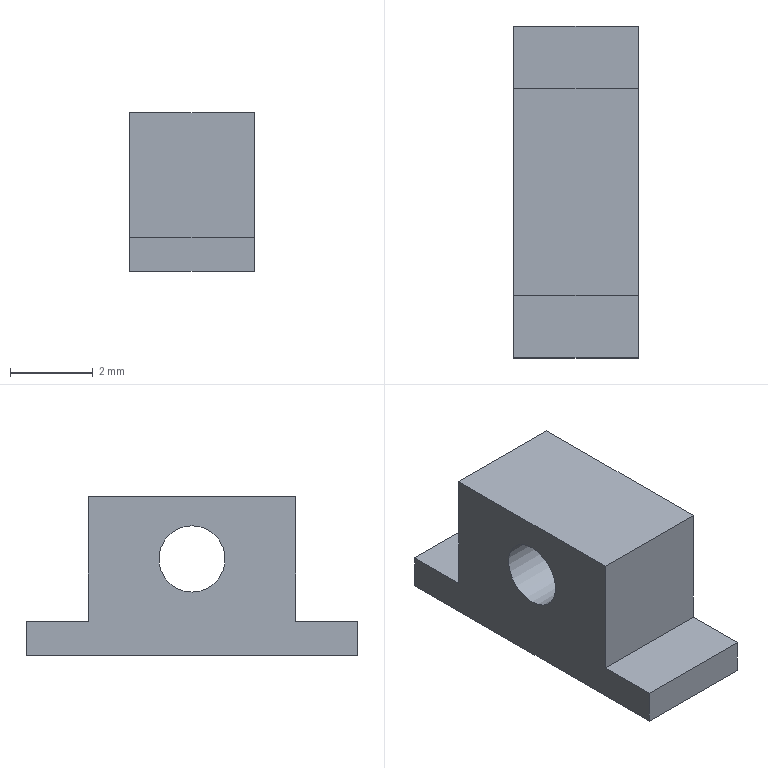Component | NX | LOWER_FIXED_SHAFT | 1 solid | 11 faces | box 3 x 8 x 3.82 mm | volume 59 mm3 | plane 10 | cylinder 1 | commonest cylinder face diameters 1.6 x1
STEP:
#1=CARTESIAN_POINT('',(0.,0.,0.));
#2=DIRECTION('',(0.,0.,1.));
#3=DIRECTION('',(1.,0.,0.));
#4=AXIS2_PLACEMENT_3D('',#1,#2,#3);
#5=CARTESIAN_POINT('',(-42.5,-2.575,4.822));
#6=VERTEX_POINT('',#5);
#7=CARTESIAN_POINT('',(-42.5,-2.575,4.));
#8=VERTEX_POINT('',#7);
#9=CARTESIAN_POINT('',(-42.5,-2.575,4.822));
#10=DIRECTION('',(0.,0.,-1.));
#11=VECTOR('',#10,1.);
#12=LINE('',#9,#11);
#13=CARTESIAN_POINT('',(-34.5,-2.575,4.822));
#14=DIRECTION('',(0.,1.,0.));
#15=DIRECTION('',(0.,0.,1.));
#16=AXIS2_PLACEMENT_3D('',#13,#14,#15);
#17=PLANE('',#16);
#18=CARTESIAN_POINT('',(0.,-8.));
#19=DIRECTION('',(-1.,0.));
#20=VECTOR('',#19,1.);
#21=LINE('',#18,#20);
#22=(GEOMETRIC_REPRESENTATION_CONTEXT(2)PARAMETRIC_REPRESENTATION_CONTEXT()REPRESENTATION_CONTEXT('',''));
#23=DEFINITIONAL_REPRESENTATION('',(#21),#22);
#24=PCURVE('',#17,#23);
#25=CARTESIAN_POINT('',(-42.5,1.425,4.822));
#26=DIRECTION('',(1.,0.,0.));
#27=DIRECTION('',(0.,0.,-1.));
#28=AXIS2_PLACEMENT_3D('',#25,#26,#27);
#29=PLANE('',#28);
#30=CARTESIAN_POINT('',(0.,-4.));
#31=DIRECTION('',(1.,0.));
#32=VECTOR('',#31,1.);
#33=LINE('',#30,#32);
#34=(GEOMETRIC_REPRESENTATION_CONTEXT(2)PARAMETRIC_REPRESENTATION_CONTEXT()REPRESENTATION_CONTEXT('',''));
#35=DEFINITIONAL_REPRESENTATION('',(#33),#34);
#36=PCURVE('',#29,#35);
#37=SURFACE_CURVE('',#12,(#24,#36),.PCURVE_S1.);
#38=EDGE_CURVE('',#6,#8,#37,.T.);
#39=ORIENTED_EDGE('',*,*,#38,.T.);
#40=CARTESIAN_POINT('',(-39.5,-2.575,4.));
#41=VERTEX_POINT('',#40);
#42=CARTESIAN_POINT('',(-34.5,-2.575,4.));
#43=DIRECTION('',(-1.,0.,0.));
#44=VECTOR('',#43,1.);
#45=LINE('',#42,#44);
#46=CARTESIAN_POINT('',(-0.8222,0.));
#47=DIRECTION('',(0.,-1.));
#48=VECTOR('',#47,1.);
#49=LINE('',#46,#48);
#50=(GEOMETRIC_REPRESENTATION_CONTEXT(2)PARAMETRIC_REPRESENTATION_CONTEXT()REPRESENTATION_CONTEXT('',''));
#51=DEFINITIONAL_REPRESENTATION('',(#49),#50);
#52=PCURVE('',#17,#51);
#53=CARTESIAN_POINT('',(-34.5,1.425,4.));
#54=DIRECTION('',(0.,0.,1.));
#55=DIRECTION('',(0.,-1.,0.));
#56=AXIS2_PLACEMENT_3D('',#53,#54,#55);
#57=PLANE('',#56);
#58=CARTESIAN_POINT('',(4.,0.));
#59=DIRECTION('',(0.,-1.));
#60=VECTOR('',#59,1.);
#61=LINE('',#58,#60);
#62=(GEOMETRIC_REPRESENTATION_CONTEXT(2)PARAMETRIC_REPRESENTATION_CONTEXT()REPRESENTATION_CONTEXT('',''));
#63=DEFINITIONAL_REPRESENTATION('',(#61),#62);
#64=PCURVE('',#57,#63);
#65=SURFACE_CURVE('',#45,(#52,#64),.PCURVE_S1.);
#66=EDGE_CURVE('',#41,#8,#65,.T.);
#67=ORIENTED_EDGE('',*,*,#66,.F.);
#68=CARTESIAN_POINT('',(-39.5,-2.575,4.822));
#69=VERTEX_POINT('',#68);
#70=CARTESIAN_POINT('',(-39.5,-2.575,4.822));
#71=DIRECTION('',(0.,0.,-1.));
#72=VECTOR('',#71,1.);
#73=LINE('',#70,#72);
#74=CARTESIAN_POINT('',(0.,-5.));
#75=DIRECTION('',(-1.,0.));
#76=VECTOR('',#75,1.);
#77=LINE('',#74,#76);
#78=(GEOMETRIC_REPRESENTATION_CONTEXT(2)PARAMETRIC_REPRESENTATION_CONTEXT()REPRESENTATION_CONTEXT('',''));
#79=DEFINITIONAL_REPRESENTATION('',(#77),#78);
#80=PCURVE('',#17,#79);
#81=CARTESIAN_POINT('',(-39.5,1.425,4.822));
#82=DIRECTION('',(1.,0.,0.));
#83=DIRECTION('',(0.,0.,-1.));
#84=AXIS2_PLACEMENT_3D('',#81,#82,#83);
#85=PLANE('',#84);
#86=CARTESIAN_POINT('',(0.,-4.));
#87=DIRECTION('',(1.,0.));
#88=VECTOR('',#87,1.);
#89=LINE('',#86,#88);
#90=(GEOMETRIC_REPRESENTATION_CONTEXT(2)PARAMETRIC_REPRESENTATION_CONTEXT()REPRESENTATION_CONTEXT('',''));
#91=DEFINITIONAL_REPRESENTATION('',(#89),#90);
#92=PCURVE('',#85,#91);
#93=SURFACE_CURVE('',#73,(#80,#92),.PCURVE_S1.);
#94=EDGE_CURVE('',#69,#41,#93,.T.);
#95=ORIENTED_EDGE('',*,*,#94,.F.);
#96=CARTESIAN_POINT('',(-34.5,-2.575,4.822));
#97=DIRECTION('',(-1.,0.,0.));
#98=VECTOR('',#97,1.);
#99=LINE('',#96,#98);
#100=CARTESIAN_POINT('',(0.,0.));
#101=DIRECTION('',(0.,-1.));
#102=VECTOR('',#101,1.);
#103=LINE('',#100,#102);
#104=(GEOMETRIC_REPRESENTATION_CONTEXT(2)PARAMETRIC_REPRESENTATION_CONTEXT()REPRESENTATION_CONTEXT('',''));
#105=DEFINITIONAL_REPRESENTATION('',(#103),#104);
#106=PCURVE('',#17,#105);
#107=CARTESIAN_POINT('',(-34.5,-1.075,4.822));
#108=DIRECTION('',(0.,0.,-1.));
#109=DIRECTION('',(0.,1.,0.));
#110=AXIS2_PLACEMENT_3D('',#107,#108,#109);
#111=PLANE('',#110);
#112=CARTESIAN_POINT('',(-1.5,0.));
#113=DIRECTION('',(0.,-1.));
#114=VECTOR('',#113,1.);
#115=LINE('',#112,#114);
#116=(GEOMETRIC_REPRESENTATION_CONTEXT(2)PARAMETRIC_REPRESENTATION_CONTEXT()REPRESENTATION_CONTEXT('',''));
#117=DEFINITIONAL_REPRESENTATION('',(#115),#116);
#118=PCURVE('',#111,#117);
#119=SURFACE_CURVE('',#99,(#106,#118),.PCURVE_S1.);
#120=EDGE_CURVE('',#69,#6,#119,.T.);
#121=ORIENTED_EDGE('',*,*,#120,.T.);
#122=EDGE_LOOP('',(#39,#67,#95,#121));
#123=FACE_BOUND('',#122,.T.);
#124=ADVANCED_FACE('',(#123),#17,.F.);
#125=CARTESIAN_POINT('',(-42.5,5.425,4.));
#126=VERTEX_POINT('',#125);
#127=CARTESIAN_POINT('',(-42.5,1.425,4.));
#128=DIRECTION('',(0.,1.,-0.));
#129=VECTOR('',#128,1.);
#130=LINE('',#127,#129);
#131=CARTESIAN_POINT('',(0.,-8.));
#132=DIRECTION('',(-1.,0.));
#133=VECTOR('',#132,1.);
#134=LINE('',#131,#133);
#135=(GEOMETRIC_REPRESENTATION_CONTEXT(2)PARAMETRIC_REPRESENTATION_CONTEXT()REPRESENTATION_CONTEXT('',''));
#136=DEFINITIONAL_REPRESENTATION('',(#134),#135);
#137=PCURVE('',#57,#136);
#138=CARTESIAN_POINT('',(0.8222,0.));
#139=DIRECTION('',(0.,1.));
#140=VECTOR('',#139,1.);
#141=LINE('',#138,#140);
#142=(GEOMETRIC_REPRESENTATION_CONTEXT(2)PARAMETRIC_REPRESENTATION_CONTEXT()REPRESENTATION_CONTEXT('',''));
#143=DEFINITIONAL_REPRESENTATION('',(#141),#142);
#144=PCURVE('',#29,#143);
#145=SURFACE_CURVE('',#130,(#137,#144),.PCURVE_S1.);
#146=EDGE_CURVE('',#8,#126,#145,.T.);
#147=ORIENTED_EDGE('',*,*,#146,.T.);
#148=CARTESIAN_POINT('',(-39.5,5.425,4.));
#149=VERTEX_POINT('',#148);
#150=CARTESIAN_POINT('',(-34.5,5.425,4.));
#151=DIRECTION('',(-1.,0.,0.));
#152=VECTOR('',#151,1.);
#153=LINE('',#150,#152);
#154=CARTESIAN_POINT('',(-4.,0.));
#155=DIRECTION('',(0.,-1.));
#156=VECTOR('',#155,1.);
#157=LINE('',#154,#156);
#158=(GEOMETRIC_REPRESENTATION_CONTEXT(2)PARAMETRIC_REPRESENTATION_CONTEXT()REPRESENTATION_CONTEXT('',''));
#159=DEFINITIONAL_REPRESENTATION('',(#157),#158);
#160=PCURVE('',#57,#159);
#161=CARTESIAN_POINT('',(-34.5,5.425,3.822));
#162=DIRECTION('',(0.,-1.,0.));
#163=DIRECTION('',(0.,0.,-1.));
#164=AXIS2_PLACEMENT_3D('',#161,#162,#163);
#165=PLANE('',#164);
#166=CARTESIAN_POINT('',(-0.1778,0.));
#167=DIRECTION('',(0.,-1.));
#168=VECTOR('',#167,1.);
#169=LINE('',#166,#168);
#170=(GEOMETRIC_REPRESENTATION_CONTEXT(2)PARAMETRIC_REPRESENTATION_CONTEXT()REPRESENTATION_CONTEXT('',''));
#171=DEFINITIONAL_REPRESENTATION('',(#169),#170);
#172=PCURVE('',#165,#171);
#173=SURFACE_CURVE('',#153,(#160,#172),.PCURVE_S1.);
#174=EDGE_CURVE('',#149,#126,#173,.T.);
#175=ORIENTED_EDGE('',*,*,#174,.F.);
#176=CARTESIAN_POINT('',(-39.5,1.425,4.));
#177=DIRECTION('',(0.,1.,-0.));
#178=VECTOR('',#177,1.);
#179=LINE('',#176,#178);
#180=CARTESIAN_POINT('',(0.,-5.));
#181=DIRECTION('',(-1.,0.));
#182=VECTOR('',#181,1.);
#183=LINE('',#180,#182);
#184=(GEOMETRIC_REPRESENTATION_CONTEXT(2)PARAMETRIC_REPRESENTATION_CONTEXT()REPRESENTATION_CONTEXT('',''));
#185=DEFINITIONAL_REPRESENTATION('',(#183),#184);
#186=PCURVE('',#57,#185);
#187=CARTESIAN_POINT('',(0.8222,0.));
#188=DIRECTION('',(0.,1.));
#189=VECTOR('',#188,1.);
#190=LINE('',#187,#189);
#191=(GEOMETRIC_REPRESENTATION_CONTEXT(2)PARAMETRIC_REPRESENTATION_CONTEXT()REPRESENTATION_CONTEXT('',''));
#192=DEFINITIONAL_REPRESENTATION('',(#190),#191);
#193=PCURVE('',#85,#192);
#194=SURFACE_CURVE('',#179,(#186,#193),.PCURVE_S1.);
#195=EDGE_CURVE('',#41,#149,#194,.T.);
#196=ORIENTED_EDGE('',*,*,#195,.F.);
#197=ORIENTED_EDGE('',*,*,#66,.T.);
#198=EDGE_LOOP('',(#147,#175,#196,#197));
#199=FACE_BOUND('',#198,.T.);
#200=ADVANCED_FACE('',(#199),#57,.F.);
#201=CARTESIAN_POINT('',(-42.5,5.425,4.822));
#202=VERTEX_POINT('',#201);
#203=CARTESIAN_POINT('',(-42.5,5.425,3.822));
#204=DIRECTION('',(0.,0.,1.));
#205=VECTOR('',#204,1.);
#206=LINE('',#203,#205);
#207=CARTESIAN_POINT('',(0.,-8.));
#208=DIRECTION('',(-1.,0.));
#209=VECTOR('',#208,1.);
#210=LINE('',#207,#209);
#211=(GEOMETRIC_REPRESENTATION_CONTEXT(2)PARAMETRIC_REPRESENTATION_CONTEXT()REPRESENTATION_CONTEXT('',''));
#212=DEFINITIONAL_REPRESENTATION('',(#210),#211);
#213=PCURVE('',#165,#212);
#214=CARTESIAN_POINT('',(1.,4.));
#215=DIRECTION('',(-1.,0.));
#216=VECTOR('',#215,1.);
#217=LINE('',#214,#216);
#218=(GEOMETRIC_REPRESENTATION_CONTEXT(2)PARAMETRIC_REPRESENTATION_CONTEXT()REPRESENTATION_CONTEXT('',''));
#219=DEFINITIONAL_REPRESENTATION('',(#217),#218);
#220=PCURVE('',#29,#219);
#221=SURFACE_CURVE('',#206,(#213,#220),.PCURVE_S1.);
#222=EDGE_CURVE('',#126,#202,#221,.T.);
#223=ORIENTED_EDGE('',*,*,#222,.T.);
#224=CARTESIAN_POINT('',(-39.5,5.425,4.822));
#225=VERTEX_POINT('',#224);
#226=CARTESIAN_POINT('',(-34.5,5.425,4.822));
#227=DIRECTION('',(-1.,0.,0.));
#228=VECTOR('',#227,1.);
#229=LINE('',#226,#228);
#230=CARTESIAN_POINT('',(-1.,0.));
#231=DIRECTION('',(0.,-1.));
#232=VECTOR('',#231,1.);
#233=LINE('',#230,#232);
#234=(GEOMETRIC_REPRESENTATION_CONTEXT(2)PARAMETRIC_REPRESENTATION_CONTEXT()REPRESENTATION_CONTEXT('',''));
#235=DEFINITIONAL_REPRESENTATION('',(#233),#234);
#236=PCURVE('',#165,#235);
#237=CARTESIAN_POINT('',(-34.5,5.425,4.822));
#238=DIRECTION('',(0.,-0.,-1.));
#239=DIRECTION('',(0.,1.,-0.));
#240=AXIS2_PLACEMENT_3D('',#237,#238,#239);
#241=PLANE('',#240);
#242=CARTESIAN_POINT('',(0.,0.));
#243=DIRECTION('',(0.,-1.));
#244=VECTOR('',#243,1.);
#245=LINE('',#242,#244);
#246=(GEOMETRIC_REPRESENTATION_CONTEXT(2)PARAMETRIC_REPRESENTATION_CONTEXT()REPRESENTATION_CONTEXT('',''));
#247=DEFINITIONAL_REPRESENTATION('',(#245),#246);
#248=PCURVE('',#241,#247);
#249=SURFACE_CURVE('',#229,(#236,#248),.PCURVE_S1.);
#250=EDGE_CURVE('',#225,#202,#249,.T.);
#251=ORIENTED_EDGE('',*,*,#250,.F.);
#252=CARTESIAN_POINT('',(-39.5,5.425,3.822));
#253=DIRECTION('',(0.,0.,1.));
#254=VECTOR('',#253,1.);
#255=LINE('',#252,#254);
#256=CARTESIAN_POINT('',(0.,-5.));
#257=DIRECTION('',(-1.,0.));
#258=VECTOR('',#257,1.);
#259=LINE('',#256,#258);
#260=(GEOMETRIC_REPRESENTATION_CONTEXT(2)PARAMETRIC_REPRESENTATION_CONTEXT()REPRESENTATION_CONTEXT('',''));
#261=DEFINITIONAL_REPRESENTATION('',(#259),#260);
#262=PCURVE('',#165,#261);
#263=CARTESIAN_POINT('',(1.,4.));
#264=DIRECTION('',(-1.,0.));
#265=VECTOR('',#264,1.);
#266=LINE('',#263,#265);
#267=(GEOMETRIC_REPRESENTATION_CONTEXT(2)PARAMETRIC_REPRESENTATION_CONTEXT()REPRESENTATION_CONTEXT('',''));
#268=DEFINITIONAL_REPRESENTATION('',(#266),#267);
#269=PCURVE('',#85,#268);
#270=SURFACE_CURVE('',#255,(#262,#269),.PCURVE_S1.);
#271=EDGE_CURVE('',#149,#225,#270,.T.);
#272=ORIENTED_EDGE('',*,*,#271,.F.);
#273=ORIENTED_EDGE('',*,*,#174,.T.);
#274=EDGE_LOOP('',(#223,#251,#272,#273));
#275=FACE_BOUND('',#274,.T.);
#276=ADVANCED_FACE('',(#275),#165,.F.);
#277=CARTESIAN_POINT('',(-42.5,3.925,4.822));
#278=VERTEX_POINT('',#277);
#279=CARTESIAN_POINT('',(-42.5,5.425,4.822));
#280=DIRECTION('',(0.,-1.,0.));
#281=VECTOR('',#280,1.);
#282=LINE('',#279,#281);
#283=CARTESIAN_POINT('',(0.,-8.));
#284=DIRECTION('',(-1.,0.));
#285=VECTOR('',#284,1.);
#286=LINE('',#283,#285);
#287=(GEOMETRIC_REPRESENTATION_CONTEXT(2)PARAMETRIC_REPRESENTATION_CONTEXT()REPRESENTATION_CONTEXT('',''));
#288=DEFINITIONAL_REPRESENTATION('',(#286),#287);
#289=PCURVE('',#241,#288);
#290=CARTESIAN_POINT('',(0.,4.));
#291=DIRECTION('',(-0.,-1.));
#292=VECTOR('',#291,1.);
#293=LINE('',#290,#292);
#294=(GEOMETRIC_REPRESENTATION_CONTEXT(2)PARAMETRIC_REPRESENTATION_CONTEXT()REPRESENTATION_CONTEXT('',''));
#295=DEFINITIONAL_REPRESENTATION('',(#293),#294);
#296=PCURVE('',#29,#295);
#297=SURFACE_CURVE('',#282,(#289,#296),.PCURVE_S1.);
#298=EDGE_CURVE('',#202,#278,#297,.T.);
#299=ORIENTED_EDGE('',*,*,#298,.T.);
#300=CARTESIAN_POINT('',(-39.5,3.925,4.822));
#301=VERTEX_POINT('',#300);
#302=CARTESIAN_POINT('',(-34.5,3.925,4.822));
#303=DIRECTION('',(-1.,0.,0.));
#304=VECTOR('',#303,1.);
#305=LINE('',#302,#304);
#306=CARTESIAN_POINT('',(-1.5,0.));
#307=DIRECTION('',(0.,-1.));
#308=VECTOR('',#307,1.);
#309=LINE('',#306,#308);
#310=(GEOMETRIC_REPRESENTATION_CONTEXT(2)PARAMETRIC_REPRESENTATION_CONTEXT()REPRESENTATION_CONTEXT('',''));
#311=DEFINITIONAL_REPRESENTATION('',(#309),#310);
#312=PCURVE('',#241,#311);
#313=CARTESIAN_POINT('',(-34.5,3.925,4.822));
#314=DIRECTION('',(0.,-1.,0.));
#315=DIRECTION('',(0.,0.,-1.));
#316=AXIS2_PLACEMENT_3D('',#313,#314,#315);
#317=PLANE('',#316);
#318=CARTESIAN_POINT('',(0.,0.));
#319=DIRECTION('',(0.,-1.));
#320=VECTOR('',#319,1.);
#321=LINE('',#318,#320);
#322=(GEOMETRIC_REPRESENTATION_CONTEXT(2)PARAMETRIC_REPRESENTATION_CONTEXT()REPRESENTATION_CONTEXT('',''));
#323=DEFINITIONAL_REPRESENTATION('',(#321),#322);
#324=PCURVE('',#317,#323);
#325=SURFACE_CURVE('',#305,(#312,#324),.PCURVE_S1.);
#326=EDGE_CURVE('',#301,#278,#325,.T.);
#327=ORIENTED_EDGE('',*,*,#326,.F.);
#328=CARTESIAN_POINT('',(-39.5,5.425,4.822));
#329=DIRECTION('',(0.,-1.,0.));
#330=VECTOR('',#329,1.);
#331=LINE('',#328,#330);
#332=CARTESIAN_POINT('',(0.,-5.));
#333=DIRECTION('',(-1.,0.));
#334=VECTOR('',#333,1.);
#335=LINE('',#332,#334);
#336=(GEOMETRIC_REPRESENTATION_CONTEXT(2)PARAMETRIC_REPRESENTATION_CONTEXT()REPRESENTATION_CONTEXT('',''));
#337=DEFINITIONAL_REPRESENTATION('',(#335),#336);
#338=PCURVE('',#241,#337);
#339=CARTESIAN_POINT('',(0.,4.));
#340=DIRECTION('',(-0.,-1.));
#341=VECTOR('',#340,1.);
#342=LINE('',#339,#341);
#343=(GEOMETRIC_REPRESENTATION_CONTEXT(2)PARAMETRIC_REPRESENTATION_CONTEXT()REPRESENTATION_CONTEXT('',''));
#344=DEFINITIONAL_REPRESENTATION('',(#342),#343);
#345=PCURVE('',#85,#344);
#346=SURFACE_CURVE('',#331,(#338,#345),.PCURVE_S1.);
#347=EDGE_CURVE('',#225,#301,#346,.T.);
#348=ORIENTED_EDGE('',*,*,#347,.F.);
#349=ORIENTED_EDGE('',*,*,#250,.T.);
#350=EDGE_LOOP('',(#299,#327,#348,#349));
#351=FACE_BOUND('',#350,.T.);
#352=ADVANCED_FACE('',(#351),#241,.F.);
#353=CARTESIAN_POINT('',(-42.5,3.925,7.822));
#354=VERTEX_POINT('',#353);
#355=CARTESIAN_POINT('',(-42.5,3.925,4.822));
#356=DIRECTION('',(0.,0.,1.));
#357=VECTOR('',#356,1.);
#358=LINE('',#355,#357);
#359=CARTESIAN_POINT('',(0.,-8.));
#360=DIRECTION('',(-1.,0.));
#361=VECTOR('',#360,1.);
#362=LINE('',#359,#361);
#363=(GEOMETRIC_REPRESENTATION_CONTEXT(2)PARAMETRIC_REPRESENTATION_CONTEXT()REPRESENTATION_CONTEXT('',''));
#364=DEFINITIONAL_REPRESENTATION('',(#362),#363);
#365=PCURVE('',#317,#364);
#366=CARTESIAN_POINT('',(0.,2.5));
#367=DIRECTION('',(-1.,0.));
#368=VECTOR('',#367,1.);
#369=LINE('',#366,#368);
#370=(GEOMETRIC_REPRESENTATION_CONTEXT(2)PARAMETRIC_REPRESENTATION_CONTEXT()REPRESENTATION_CONTEXT('',''));
#371=DEFINITIONAL_REPRESENTATION('',(#369),#370);
#372=PCURVE('',#29,#371);
#373=SURFACE_CURVE('',#358,(#365,#372),.PCURVE_S1.);
#374=EDGE_CURVE('',#278,#354,#373,.T.);
#375=ORIENTED_EDGE('',*,*,#374,.T.);
#376=CARTESIAN_POINT('',(-39.5,3.925,7.822));
#377=VERTEX_POINT('',#376);
#378=CARTESIAN_POINT('',(-34.5,3.925,7.822));
#379=DIRECTION('',(-1.,0.,0.));
#380=VECTOR('',#379,1.);
#381=LINE('',#378,#380);
#382=CARTESIAN_POINT('',(-3.,0.));
#383=DIRECTION('',(0.,-1.));
#384=VECTOR('',#383,1.);
#385=LINE('',#382,#384);
#386=(GEOMETRIC_REPRESENTATION_CONTEXT(2)PARAMETRIC_REPRESENTATION_CONTEXT()REPRESENTATION_CONTEXT('',''));
#387=DEFINITIONAL_REPRESENTATION('',(#385),#386);
#388=PCURVE('',#317,#387);
#389=CARTESIAN_POINT('',(-34.5,1.425,7.822));
#390=DIRECTION('',(0.,0.,-1.));
#391=DIRECTION('',(0.,1.,0.));
#392=AXIS2_PLACEMENT_3D('',#389,#390,#391);
#393=PLANE('',#392);
#394=CARTESIAN_POINT('',(2.5,0.));
#395=DIRECTION('',(0.,-1.));
#396=VECTOR('',#395,1.);
#397=LINE('',#394,#396);
#398=(GEOMETRIC_REPRESENTATION_CONTEXT(2)PARAMETRIC_REPRESENTATION_CONTEXT()REPRESENTATION_CONTEXT('',''));
#399=DEFINITIONAL_REPRESENTATION('',(#397),#398);
#400=PCURVE('',#393,#399);
#401=SURFACE_CURVE('',#381,(#388,#400),.PCURVE_S1.);
#402=EDGE_CURVE('',#377,#354,#401,.T.);
#403=ORIENTED_EDGE('',*,*,#402,.F.);
#404=CARTESIAN_POINT('',(-39.5,3.925,4.822));
#405=DIRECTION('',(0.,0.,1.));
#406=VECTOR('',#405,1.);
#407=LINE('',#404,#406);
#408=CARTESIAN_POINT('',(0.,-5.));
#409=DIRECTION('',(-1.,0.));
#410=VECTOR('',#409,1.);
#411=LINE('',#408,#410);
#412=(GEOMETRIC_REPRESENTATION_CONTEXT(2)PARAMETRIC_REPRESENTATION_CONTEXT()REPRESENTATION_CONTEXT('',''));
#413=DEFINITIONAL_REPRESENTATION('',(#411),#412);
#414=PCURVE('',#317,#413);
#415=CARTESIAN_POINT('',(0.,2.5));
#416=DIRECTION('',(-1.,0.));
#417=VECTOR('',#416,1.);
#418=LINE('',#415,#417);
#419=(GEOMETRIC_REPRESENTATION_CONTEXT(2)PARAMETRIC_REPRESENTATION_CONTEXT()REPRESENTATION_CONTEXT('',''));
#420=DEFINITIONAL_REPRESENTATION('',(#418),#419);
#421=PCURVE('',#85,#420);
#422=SURFACE_CURVE('',#407,(#414,#421),.PCURVE_S1.);
#423=EDGE_CURVE('',#301,#377,#422,.T.);
#424=ORIENTED_EDGE('',*,*,#423,.F.);
#425=ORIENTED_EDGE('',*,*,#326,.T.);
#426=EDGE_LOOP('',(#375,#403,#424,#425));
#427=FACE_BOUND('',#426,.T.);
#428=ADVANCED_FACE('',(#427),#317,.F.);
#429=CARTESIAN_POINT('',(-42.5,-1.075,7.822));
#430=VERTEX_POINT('',#429);
#431=CARTESIAN_POINT('',(-42.5,1.425,7.822));
#432=DIRECTION('',(0.,-1.,-0.));
#433=VECTOR('',#432,1.);
#434=LINE('',#431,#433);
#435=CARTESIAN_POINT('',(0.,-8.));
#436=DIRECTION('',(-1.,0.));
#437=VECTOR('',#436,1.);
#438=LINE('',#435,#437);
#439=(GEOMETRIC_REPRESENTATION_CONTEXT(2)PARAMETRIC_REPRESENTATION_CONTEXT()REPRESENTATION_CONTEXT('',''));
#440=DEFINITIONAL_REPRESENTATION('',(#438),#439);
#441=PCURVE('',#393,#440);
#442=CARTESIAN_POINT('',(-3.,0.));
#443=DIRECTION('',(0.,-1.));
#444=VECTOR('',#443,1.);
#445=LINE('',#442,#444);
#446=(GEOMETRIC_REPRESENTATION_CONTEXT(2)PARAMETRIC_REPRESENTATION_CONTEXT()REPRESENTATION_CONTEXT('',''));
#447=DEFINITIONAL_REPRESENTATION('',(#445),#446);
#448=PCURVE('',#29,#447);
#449=SURFACE_CURVE('',#434,(#441,#448),.PCURVE_S1.);
#450=EDGE_CURVE('',#354,#430,#449,.T.);
#451=ORIENTED_EDGE('',*,*,#450,.T.);
#452=CARTESIAN_POINT('',(-39.5,-1.075,7.822));
#453=VERTEX_POINT('',#452);
#454=CARTESIAN_POINT('',(-34.5,-1.075,7.822));
#455=DIRECTION('',(-1.,0.,0.));
#456=VECTOR('',#455,1.);
#457=LINE('',#454,#456);
#458=CARTESIAN_POINT('',(-2.5,0.));
#459=DIRECTION('',(0.,-1.));
#460=VECTOR('',#459,1.);
#461=LINE('',#458,#460);
#462=(GEOMETRIC_REPRESENTATION_CONTEXT(2)PARAMETRIC_REPRESENTATION_CONTEXT()REPRESENTATION_CONTEXT('',''));
#463=DEFINITIONAL_REPRESENTATION('',(#461),#462);
#464=PCURVE('',#393,#463);
#465=CARTESIAN_POINT('',(-34.5,-1.075,7.822));
#466=DIRECTION('',(0.,1.,0.));
#467=DIRECTION('',(0.,0.,1.));
#468=AXIS2_PLACEMENT_3D('',#465,#466,#467);
#469=PLANE('',#468);
#470=CARTESIAN_POINT('',(0.,0.));
#471=DIRECTION('',(0.,-1.));
#472=VECTOR('',#471,1.);
#473=LINE('',#470,#472);
#474=(GEOMETRIC_REPRESENTATION_CONTEXT(2)PARAMETRIC_REPRESENTATION_CONTEXT()REPRESENTATION_CONTEXT('',''));
#475=DEFINITIONAL_REPRESENTATION('',(#473),#474);
#476=PCURVE('',#469,#475);
#477=SURFACE_CURVE('',#457,(#464,#476),.PCURVE_S1.);
#478=EDGE_CURVE('',#453,#430,#477,.T.);
#479=ORIENTED_EDGE('',*,*,#478,.F.);
#480=CARTESIAN_POINT('',(-39.5,3.925,7.822));
#481=DIRECTION('',(0.,-1.,0.));
#482=VECTOR('',#481,1.);
#483=LINE('',#480,#482);
#484=CARTESIAN_POINT('',(2.5,-5.));
#485=DIRECTION('',(-1.,0.));
#486=VECTOR('',#485,1.);
#487=LINE('',#484,#486);
#488=(GEOMETRIC_REPRESENTATION_CONTEXT(2)PARAMETRIC_REPRESENTATION_CONTEXT()REPRESENTATION_CONTEXT('',''));
#489=DEFINITIONAL_REPRESENTATION('',(#487),#488);
#490=PCURVE('',#393,#489);
#491=CARTESIAN_POINT('',(-3.,2.5));
#492=DIRECTION('',(-0.,-1.));
#493=VECTOR('',#492,1.);
#494=LINE('',#491,#493);
#495=(GEOMETRIC_REPRESENTATION_CONTEXT(2)PARAMETRIC_REPRESENTATION_CONTEXT()REPRESENTATION_CONTEXT('',''));
#496=DEFINITIONAL_REPRESENTATION('',(#494),#495);
#497=PCURVE('',#85,#496);
#498=SURFACE_CURVE('',#483,(#490,#497),.PCURVE_S1.);
#499=EDGE_CURVE('',#377,#453,#498,.T.);
#500=ORIENTED_EDGE('',*,*,#499,.F.);
#501=ORIENTED_EDGE('',*,*,#402,.T.);
#502=EDGE_LOOP('',(#451,#479,#500,#501));
#503=FACE_BOUND('',#502,.T.);
#504=ADVANCED_FACE('',(#503),#393,.F.);
#505=CARTESIAN_POINT('',(-42.5,-1.075,4.822));
#506=VERTEX_POINT('',#505);
#507=CARTESIAN_POINT('',(-42.5,-1.075,7.822));
#508=DIRECTION('',(0.,0.,-1.));
#509=VECTOR('',#508,1.);
#510=LINE('',#507,#509);
#511=CARTESIAN_POINT('',(0.,-8.));
#512=DIRECTION('',(-1.,0.));
#513=VECTOR('',#512,1.);
#514=LINE('',#511,#513);
#515=(GEOMETRIC_REPRESENTATION_CONTEXT(2)PARAMETRIC_REPRESENTATION_CONTEXT()REPRESENTATION_CONTEXT('',''));
#516=DEFINITIONAL_REPRESENTATION('',(#514),#515);
#517=PCURVE('',#469,#516);
#518=CARTESIAN_POINT('',(-3.,-2.5));
#519=DIRECTION('',(1.,0.));
#520=VECTOR('',#519,1.);
#521=LINE('',#518,#520);
#522=(GEOMETRIC_REPRESENTATION_CONTEXT(2)PARAMETRIC_REPRESENTATION_CONTEXT()REPRESENTATION_CONTEXT('',''));
#523=DEFINITIONAL_REPRESENTATION('',(#521),#522);
#524=PCURVE('',#29,#523);
#525=SURFACE_CURVE('',#510,(#517,#524),.PCURVE_S1.);
#526=EDGE_CURVE('',#430,#506,#525,.T.);
#527=ORIENTED_EDGE('',*,*,#526,.T.);
#528=CARTESIAN_POINT('',(-39.5,-1.075,4.822));
#529=VERTEX_POINT('',#528);
#530=CARTESIAN_POINT('',(-34.5,-1.075,4.822));
#531=DIRECTION('',(-1.,0.,0.));
#532=VECTOR('',#531,1.);
#533=LINE('',#530,#532);
#534=CARTESIAN_POINT('',(-3.,0.));
#535=DIRECTION('',(0.,-1.));
#536=VECTOR('',#535,1.);
#537=LINE('',#534,#536);
#538=(GEOMETRIC_REPRESENTATION_CONTEXT(2)PARAMETRIC_REPRESENTATION_CONTEXT()REPRESENTATION_CONTEXT('',''));
#539=DEFINITIONAL_REPRESENTATION('',(#537),#538);
#540=PCURVE('',#469,#539);
#541=CARTESIAN_POINT('',(0.,0.));
#542=DIRECTION('',(0.,-1.));
#543=VECTOR('',#542,1.);
#544=LINE('',#541,#543);
#545=(GEOMETRIC_REPRESENTATION_CONTEXT(2)PARAMETRIC_REPRESENTATION_CONTEXT()REPRESENTATION_CONTEXT('',''));
#546=DEFINITIONAL_REPRESENTATION('',(#544),#545);
#547=PCURVE('',#111,#546);
#548=SURFACE_CURVE('',#533,(#540,#547),.PCURVE_S1.);
#549=EDGE_CURVE('',#529,#506,#548,.T.);
#550=ORIENTED_EDGE('',*,*,#549,.F.);
#551=CARTESIAN_POINT('',(-39.5,-1.075,7.822));
#552=DIRECTION('',(0.,0.,-1.));
#553=VECTOR('',#552,1.);
#554=LINE('',#551,#553);
#555=CARTESIAN_POINT('',(0.,-5.));
#556=DIRECTION('',(-1.,0.));
#557=VECTOR('',#556,1.);
#558=LINE('',#555,#557);
#559=(GEOMETRIC_REPRESENTATION_CONTEXT(2)PARAMETRIC_REPRESENTATION_CONTEXT()REPRESENTATION_CONTEXT('',''));
#560=DEFINITIONAL_REPRESENTATION('',(#558),#559);
#561=PCURVE('',#469,#560);
#562=CARTESIAN_POINT('',(-3.,-2.5));
#563=DIRECTION('',(1.,0.));
#564=VECTOR('',#563,1.);
#565=LINE('',#562,#564);
#566=(GEOMETRIC_REPRESENTATION_CONTEXT(2)PARAMETRIC_REPRESENTATION_CONTEXT()REPRESENTATION_CONTEXT('',''));
#567=DEFINITIONAL_REPRESENTATION('',(#565),#566);
#568=PCURVE('',#85,#567);
#569=SURFACE_CURVE('',#554,(#561,#568),.PCURVE_S1.);
#570=EDGE_CURVE('',#453,#529,#569,.T.);
#571=ORIENTED_EDGE('',*,*,#570,.F.);
#572=ORIENTED_EDGE('',*,*,#478,.T.);
#573=EDGE_LOOP('',(#527,#550,#571,#572));
#574=FACE_BOUND('',#573,.T.);
#575=ADVANCED_FACE('',(#574),#469,.F.);
#576=CARTESIAN_POINT('',(-42.5,-1.075,4.822));
#577=DIRECTION('',(0.,-1.,-0.));
#578=VECTOR('',#577,1.);
#579=LINE('',#576,#578);
#580=CARTESIAN_POINT('',(0.,-8.));
#581=DIRECTION('',(-1.,0.));
#582=VECTOR('',#581,1.);
#583=LINE('',#580,#582);
#584=(GEOMETRIC_REPRESENTATION_CONTEXT(2)PARAMETRIC_REPRESENTATION_CONTEXT()REPRESENTATION_CONTEXT('',''));
#585=DEFINITIONAL_REPRESENTATION('',(#583),#584);
#586=PCURVE('',#111,#585);
#587=CARTESIAN_POINT('',(0.,-2.5));
#588=DIRECTION('',(0.,-1.));
#589=VECTOR('',#588,1.);
#590=LINE('',#587,#589);
#591=(GEOMETRIC_REPRESENTATION_CONTEXT(2)PARAMETRIC_REPRESENTATION_CONTEXT()REPRESENTATION_CONTEXT('',''));
#592=DEFINITIONAL_REPRESENTATION('',(#590),#591);
#593=PCURVE('',#29,#592);
#594=SURFACE_CURVE('',#579,(#586,#593),.PCURVE_S1.);
#595=EDGE_CURVE('',#506,#6,#594,.T.);
#596=ORIENTED_EDGE('',*,*,#595,.T.);
#597=ORIENTED_EDGE('',*,*,#120,.F.);
#598=CARTESIAN_POINT('',(-39.5,-1.075,4.822));
#599=DIRECTION('',(0.,-1.,-0.));
#600=VECTOR('',#599,1.);
#601=LINE('',#598,#600);
#602=CARTESIAN_POINT('',(0.,-5.));
#603=DIRECTION('',(-1.,0.));
#604=VECTOR('',#603,1.);
#605=LINE('',#602,#604);
#606=(GEOMETRIC_REPRESENTATION_CONTEXT(2)PARAMETRIC_REPRESENTATION_CONTEXT()REPRESENTATION_CONTEXT('',''));
#607=DEFINITIONAL_REPRESENTATION('',(#605),#606);
#608=PCURVE('',#111,#607);
#609=CARTESIAN_POINT('',(0.,-2.5));
#610=DIRECTION('',(0.,-1.));
#611=VECTOR('',#610,1.);
#612=LINE('',#609,#611);
#613=(GEOMETRIC_REPRESENTATION_CONTEXT(2)PARAMETRIC_REPRESENTATION_CONTEXT()REPRESENTATION_CONTEXT('',''));
#614=DEFINITIONAL_REPRESENTATION('',(#612),#613);
#615=PCURVE('',#85,#614);
#616=SURFACE_CURVE('',#601,(#608,#615),.PCURVE_S1.);
#617=EDGE_CURVE('',#529,#69,#616,.T.);
#618=ORIENTED_EDGE('',*,*,#617,.F.);
#619=ORIENTED_EDGE('',*,*,#549,.T.);
#620=EDGE_LOOP('',(#596,#597,#618,#619));
#621=FACE_BOUND('',#620,.T.);
#622=ADVANCED_FACE('',(#621),#111,.F.);
#623=CARTESIAN_POINT('',(-39.5,1.425,5.522));
#624=VERTEX_POINT('',#623);
#625=CARTESIAN_POINT('',(-39.5,1.425,6.322));
#626=DIRECTION('',(-1.,0.,0.));
#627=DIRECTION('',(0.,0.,-1.));
#628=AXIS2_PLACEMENT_3D('',#625,#626,#627);
#629=CIRCLE('',#628,0.8);
#630=CARTESIAN_POINT('',(-0.7,0.));
#631=CARTESIAN_POINT('',(-0.7,-1.386));
#632=CARTESIAN_POINT('',(-1.9,-0.6928));
#633=CARTESIAN_POINT('',(-3.1,-0.));
#634=CARTESIAN_POINT('',(-1.9,0.6928));
#635=CARTESIAN_POINT('',(-0.7,1.386));
#636=CARTESIAN_POINT('',(-0.7,0.));
#637=(BOUNDED_CURVE()B_SPLINE_CURVE(2,(#630,#631,#632,#633,#634,#635,#636),.UNSPECIFIED.,.T.,.F.)B_SPLINE_CURVE_WITH_KNOTS((1,2,2,2,2,1),(-2.094,0.,2.094,4.189,6.283,8.378),.UNSPECIFIED.)CURVE()GEOMETRIC_REPRESENTATION_ITEM()RATIONAL_B_SPLINE_CURVE((1.,0.5,1.,0.5,1.,0.5,1.))REPRESENTATION_ITEM(''));
#638=(GEOMETRIC_REPRESENTATION_CONTEXT(2)PARAMETRIC_REPRESENTATION_CONTEXT()REPRESENTATION_CONTEXT('',''));
#639=DEFINITIONAL_REPRESENTATION('',(#637),#638);
#640=PCURVE('',#85,#639);
#641=CARTESIAN_POINT('',(-33.7,1.425,6.322));
#642=DIRECTION('',(-1.,0.,0.));
#643=DIRECTION('',(0.,0.,1.));
#644=AXIS2_PLACEMENT_3D('',#641,#642,#643);
#645=CYLINDRICAL_SURFACE('',#644,0.8);
#646=CARTESIAN_POINT('',(3.142,5.8));
#647=DIRECTION('',(1.,0.));
#648=VECTOR('',#647,1.);
#649=LINE('',#646,#648);
#650=(GEOMETRIC_REPRESENTATION_CONTEXT(2)PARAMETRIC_REPRESENTATION_CONTEXT()REPRESENTATION_CONTEXT('',''));
#651=DEFINITIONAL_REPRESENTATION('',(#649),#650);
#652=PCURVE('',#645,#651);
#653=SURFACE_CURVE('',#629,(#640,#652),.PCURVE_S1.);
#654=EDGE_CURVE('',#624,#624,#653,.T.);
#655=ORIENTED_EDGE('',*,*,#654,.T.);
#656=EDGE_LOOP('',(#655));
#657=FACE_BOUND('',#656,.T.);
#658=ORIENTED_EDGE('',*,*,#94,.T.);
#659=ORIENTED_EDGE('',*,*,#195,.T.);
#660=ORIENTED_EDGE('',*,*,#271,.T.);
#661=ORIENTED_EDGE('',*,*,#347,.T.);
#662=ORIENTED_EDGE('',*,*,#423,.T.);
#663=ORIENTED_EDGE('',*,*,#499,.T.);
#664=ORIENTED_EDGE('',*,*,#570,.T.);
#665=ORIENTED_EDGE('',*,*,#617,.T.);
#666=EDGE_LOOP('',(#658,#659,#660,#661,#662,#663,#664,#665));
#667=FACE_BOUND('',#666,.T.);
#668=ADVANCED_FACE('',(#657,#667),#85,.T.);
#669=CARTESIAN_POINT('',(-42.5,1.425,5.522));
#670=VERTEX_POINT('',#669);
#671=CARTESIAN_POINT('',(-42.5,1.425,6.322));
#672=DIRECTION('',(-1.,0.,0.));
#673=DIRECTION('',(0.,0.,-1.));
#674=AXIS2_PLACEMENT_3D('',#671,#672,#673);
#675=CIRCLE('',#674,0.8);
#676=CARTESIAN_POINT('',(-0.7,0.));
#677=CARTESIAN_POINT('',(-0.7,-1.386));
#678=CARTESIAN_POINT('',(-1.9,-0.6928));
#679=CARTESIAN_POINT('',(-3.1,-0.));
#680=CARTESIAN_POINT('',(-1.9,0.6928));
#681=CARTESIAN_POINT('',(-0.7,1.386));
#682=CARTESIAN_POINT('',(-0.7,0.));
#683=(BOUNDED_CURVE()B_SPLINE_CURVE(2,(#676,#677,#678,#679,#680,#681,#682),.UNSPECIFIED.,.T.,.F.)B_SPLINE_CURVE_WITH_KNOTS((1,2,2,2,2,1),(-2.094,0.,2.094,4.189,6.283,8.378),.UNSPECIFIED.)CURVE()GEOMETRIC_REPRESENTATION_ITEM()RATIONAL_B_SPLINE_CURVE((1.,0.5,1.,0.5,1.,0.5,1.))REPRESENTATION_ITEM(''));
#684=(GEOMETRIC_REPRESENTATION_CONTEXT(2)PARAMETRIC_REPRESENTATION_CONTEXT()REPRESENTATION_CONTEXT('',''));
#685=DEFINITIONAL_REPRESENTATION('',(#683),#684);
#686=PCURVE('',#29,#685);
#687=CARTESIAN_POINT('',(3.142,8.8));
#688=DIRECTION('',(1.,0.));
#689=VECTOR('',#688,1.);
#690=LINE('',#687,#689);
#691=(GEOMETRIC_REPRESENTATION_CONTEXT(2)PARAMETRIC_REPRESENTATION_CONTEXT()REPRESENTATION_CONTEXT('',''));
#692=DEFINITIONAL_REPRESENTATION('',(#690),#691);
#693=PCURVE('',#645,#692);
#694=SURFACE_CURVE('',#675,(#686,#693),.PCURVE_S1.);
#695=EDGE_CURVE('',#670,#670,#694,.T.);
#696=ORIENTED_EDGE('',*,*,#695,.F.);
#697=EDGE_LOOP('',(#696));
#698=FACE_BOUND('',#697,.T.);
#699=ORIENTED_EDGE('',*,*,#38,.F.);
#700=ORIENTED_EDGE('',*,*,#595,.F.);
#701=ORIENTED_EDGE('',*,*,#526,.F.);
#702=ORIENTED_EDGE('',*,*,#450,.F.);
#703=ORIENTED_EDGE('',*,*,#374,.F.);
#704=ORIENTED_EDGE('',*,*,#298,.F.);
#705=ORIENTED_EDGE('',*,*,#222,.F.);
#706=ORIENTED_EDGE('',*,*,#146,.F.);
#707=EDGE_LOOP('',(#699,#700,#701,#702,#703,#704,#705,#706));
#708=FACE_BOUND('',#707,.T.);
#709=ADVANCED_FACE('',(#698,#708),#29,.F.);
#710=ORIENTED_EDGE('',*,*,#654,.T.);
#711=CARTESIAN_POINT('',(-39.5,1.425,5.522));
#712=CARTESIAN_POINT('',(-42.5,1.425,5.522));
#713=B_SPLINE_CURVE_WITH_KNOTS('',1,(#711,#712),.UNSPECIFIED.,.F.,.F.,(2,2),(5.8,8.8),.PIECEWISE_BEZIER_KNOTS.);
#714=CARTESIAN_POINT('',(9.425,0.));
#715=DIRECTION('',(0.,1.));
#716=VECTOR('',#715,1.);
#717=LINE('',#714,#716);
#718=(GEOMETRIC_REPRESENTATION_CONTEXT(2)PARAMETRIC_REPRESENTATION_CONTEXT()REPRESENTATION_CONTEXT('',''));
#719=DEFINITIONAL_REPRESENTATION('',(#717),#718);
#720=PCURVE('',#645,#719);
#721=CARTESIAN_POINT('',(3.142,0.));
#722=DIRECTION('',(0.,1.));
#723=VECTOR('',#722,1.);
#724=LINE('',#721,#723);
#725=(GEOMETRIC_REPRESENTATION_CONTEXT(2)PARAMETRIC_REPRESENTATION_CONTEXT()REPRESENTATION_CONTEXT('',''));
#726=DEFINITIONAL_REPRESENTATION('',(#724),#725);
#727=PCURVE('',#645,#726);
#728=SEAM_CURVE('',#713,(#720,#727),.PCURVE_S1.);
#729=EDGE_CURVE('',#624,#670,#728,.T.);
#730=ORIENTED_EDGE('',*,*,#729,.T.);
#731=ORIENTED_EDGE('',*,*,#695,.F.);
#732=ORIENTED_EDGE('',*,*,#729,.F.);
#733=EDGE_LOOP('',(#710,#730,#731,#732));
#734=FACE_BOUND('',#733,.F.);
#735=ADVANCED_FACE('',(#734),#645,.F.);
#736=CLOSED_SHELL('',(#124,#200,#276,#352,#428,#504,#575,#622,#668,#709,#735));
#737=MANIFOLD_SOLID_BREP('',#736);
#738=(LENGTH_UNIT()NAMED_UNIT(*)SI_UNIT(.MILLI.,.METRE.));
#739=UNCERTAINTY_MEASURE_WITH_UNIT(LENGTH_MEASURE(0.000001),#738,'','');
#740=(NAMED_UNIT(*)PLANE_ANGLE_UNIT()SI_UNIT($,.RADIAN.));
#741=(NAMED_UNIT(*)SI_UNIT($,.STERADIAN.)SOLID_ANGLE_UNIT());
#742=(GEOMETRIC_REPRESENTATION_CONTEXT(3)GLOBAL_UNCERTAINTY_ASSIGNED_CONTEXT((#739))GLOBAL_UNIT_ASSIGNED_CONTEXT((#738,#740,#741))REPRESENTATION_CONTEXT('',''));
#743=ADVANCED_BREP_SHAPE_REPRESENTATION('',(#4,#737),#742);